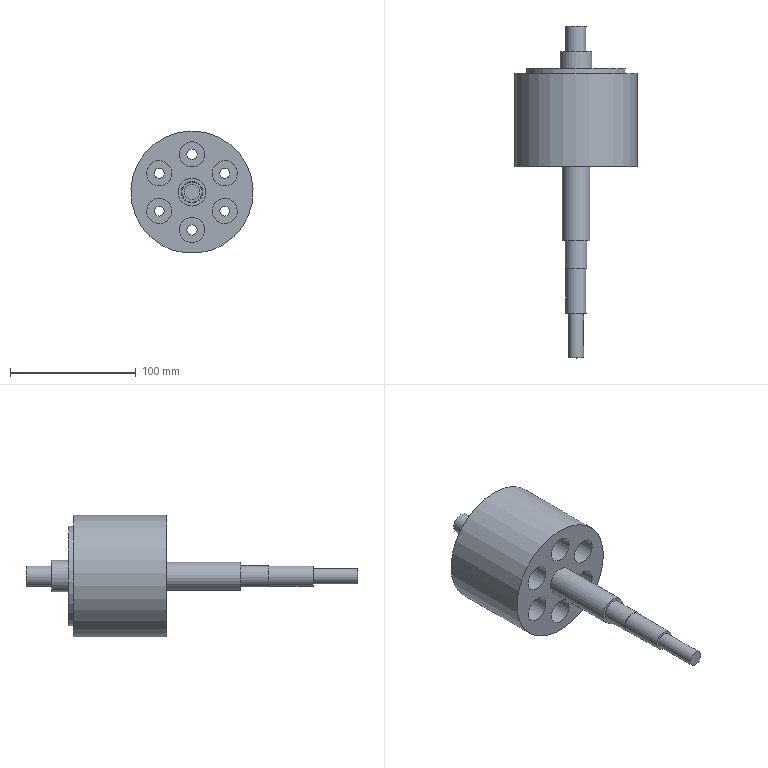Component | NX | ROTOR | 1 solid | 42 faces | volume 485879 mm3 | cylinder 23 | plane 19 | commonest cylinder face diameters 20 x6 8 x6 16 x2 4 x2 12 x1 17 x1 22 x1 97 x1